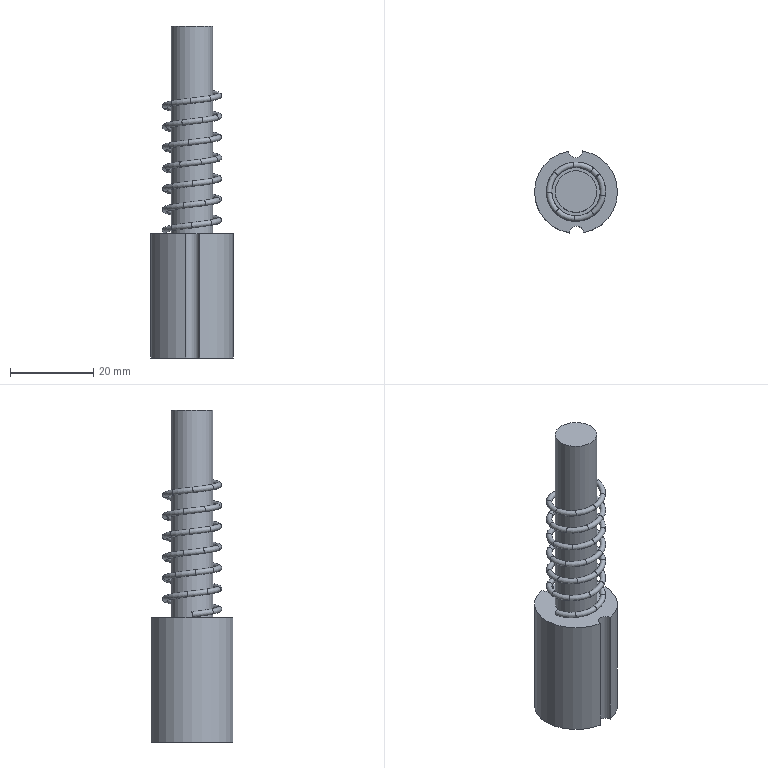Component | NX | PUNCH | 2 solids | 66 faces | volume 13434 mm3 | torus 56 | plane 5 | cylinder 5 | commonest cylinder face diameters 20 x2 3.5 x2 10 x1